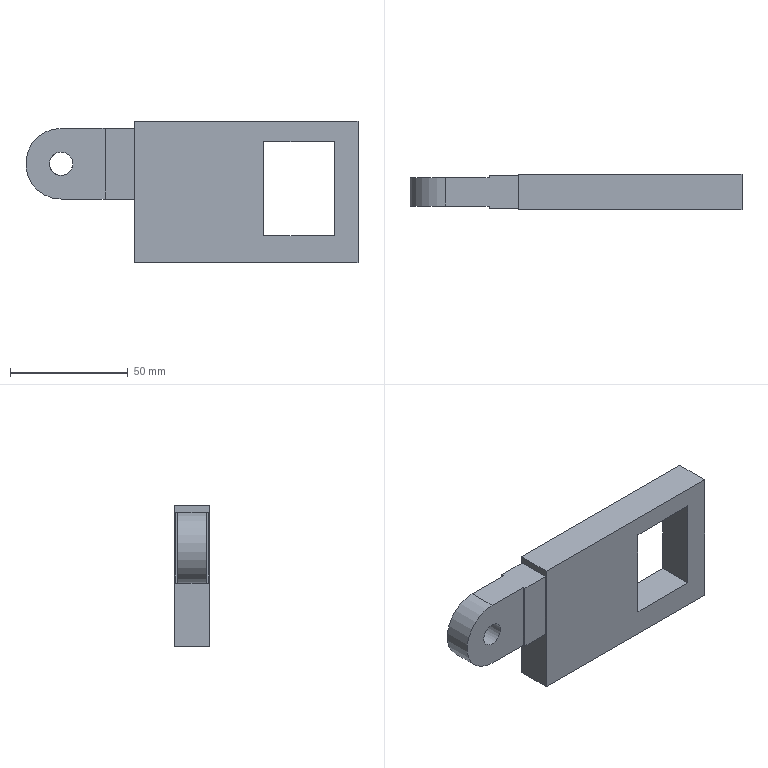Component | NX | PUSH_ROD | 1 solid | 20 faces | volume 82693 mm3 | plane 18 | cylinder 2 | commonest cylinder face diameters 30 x1 10 x1